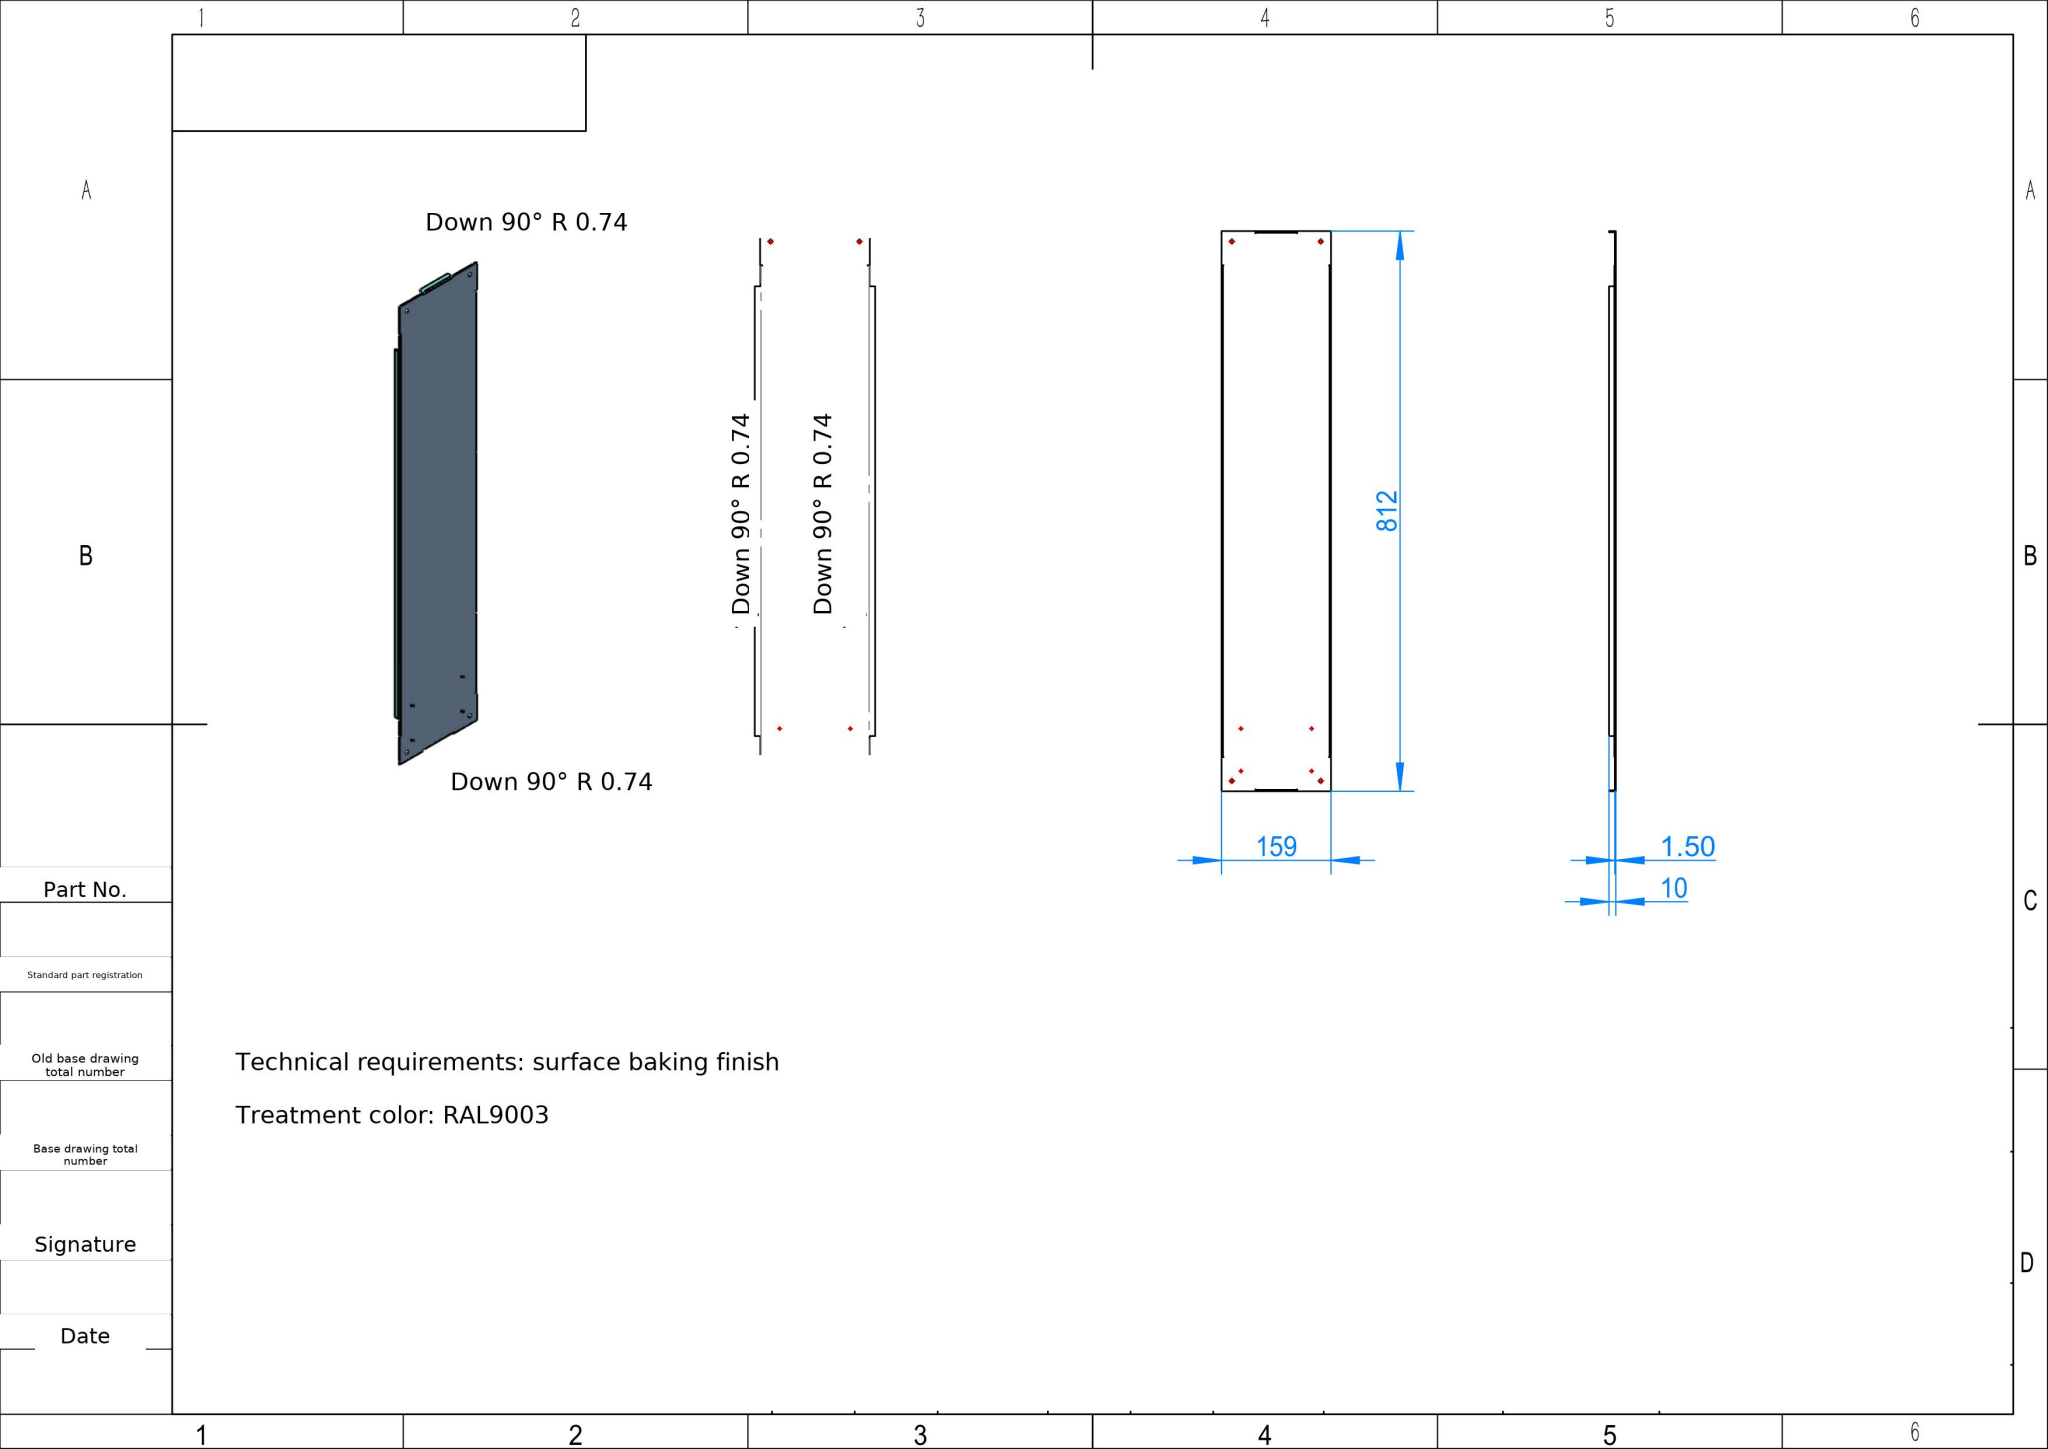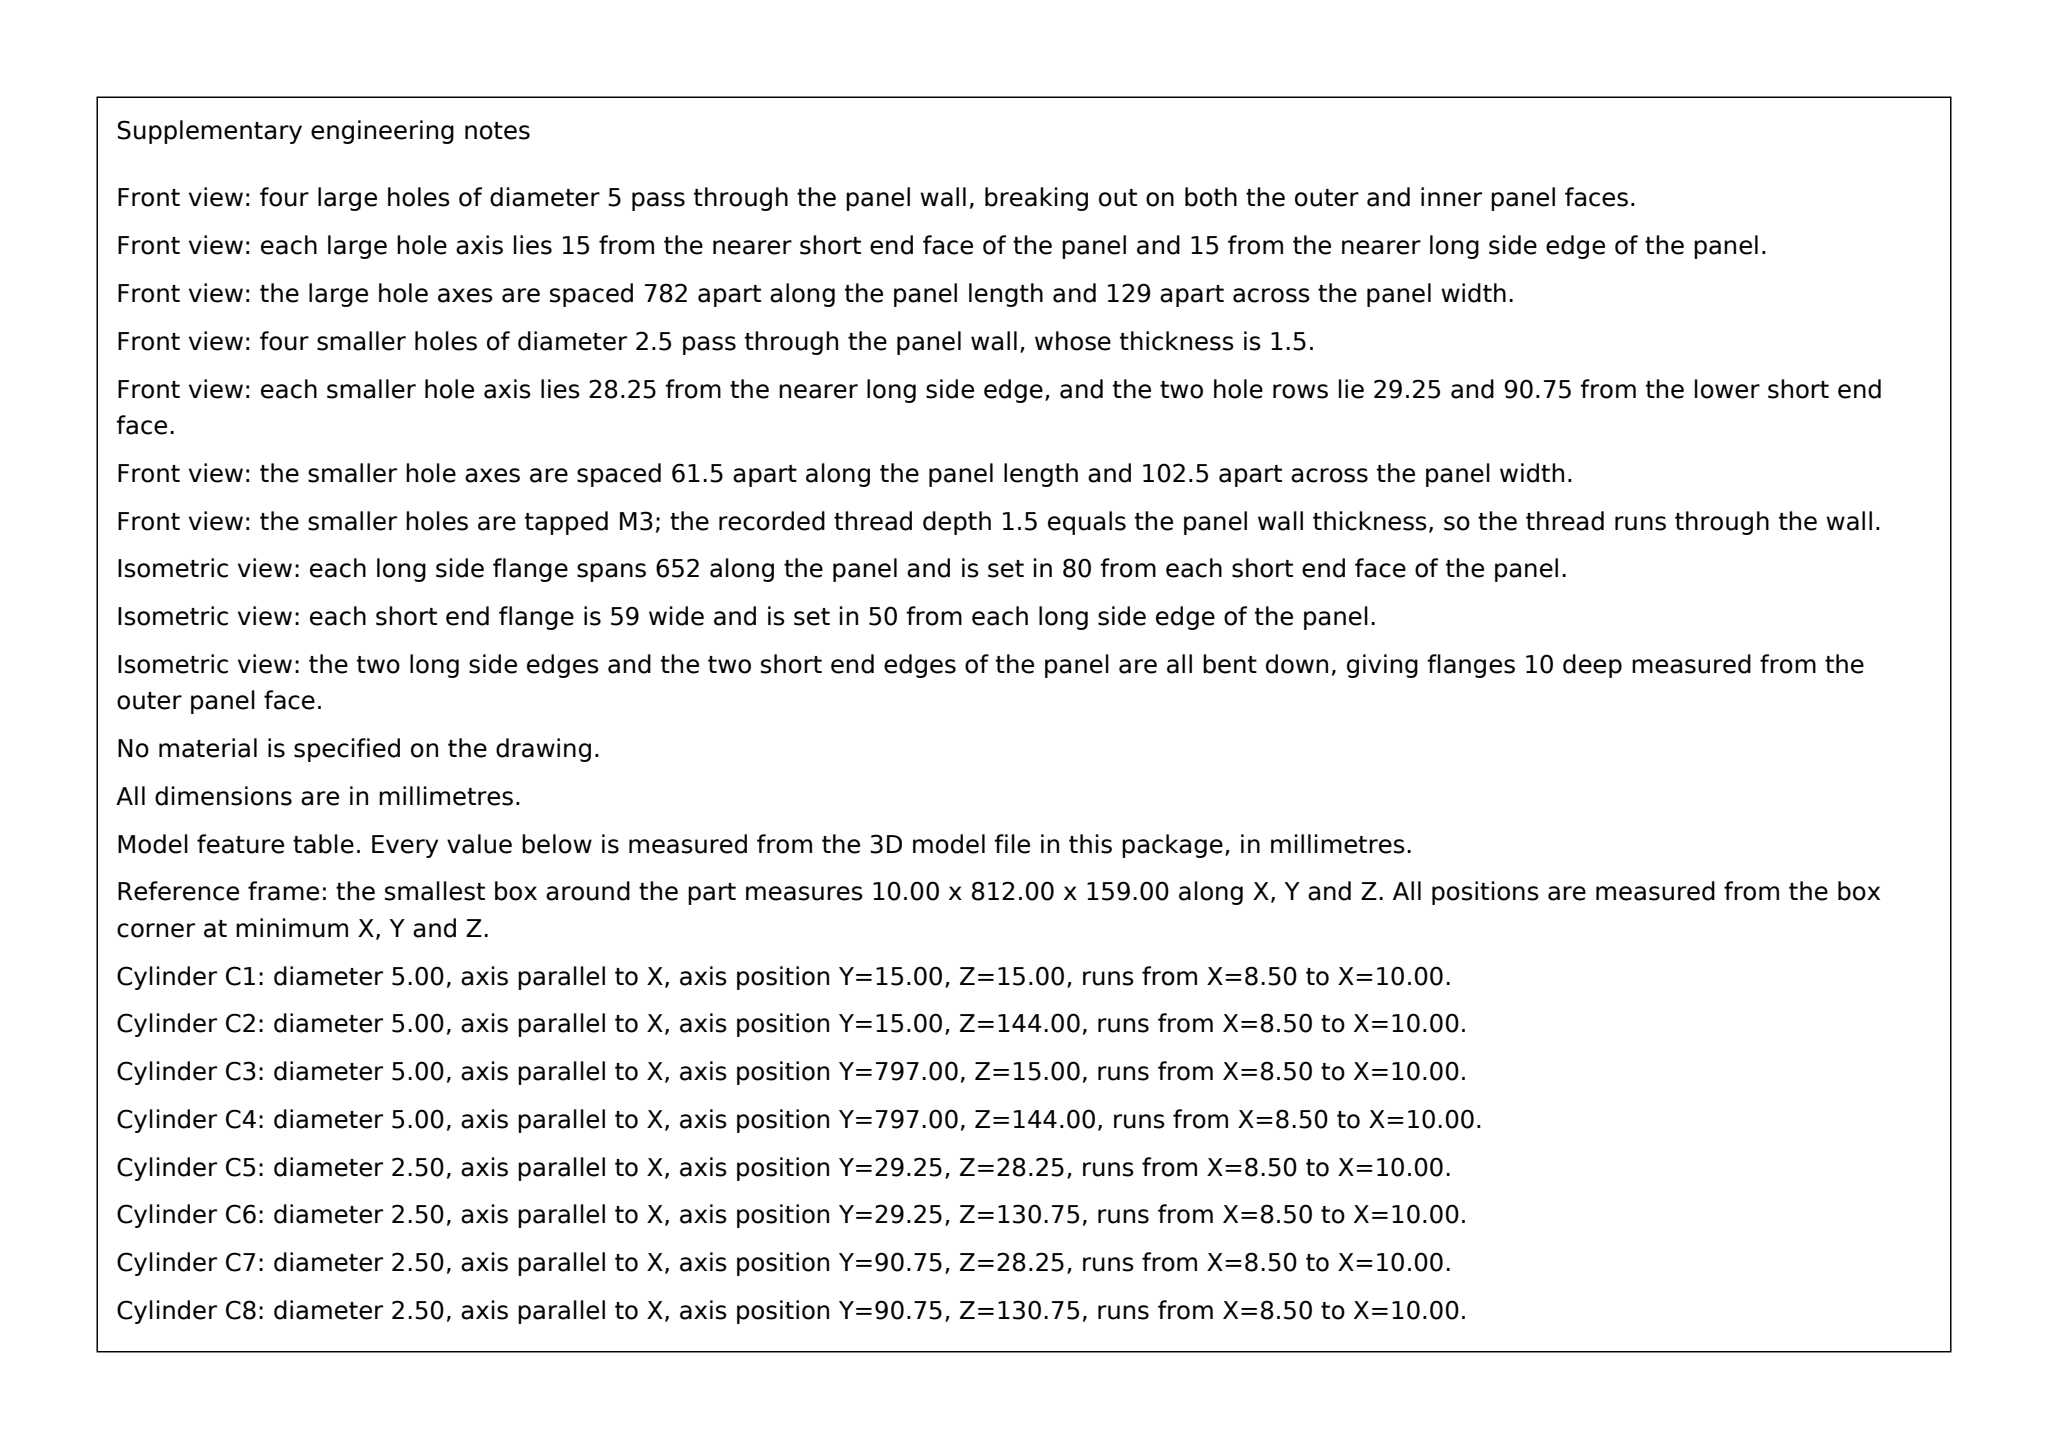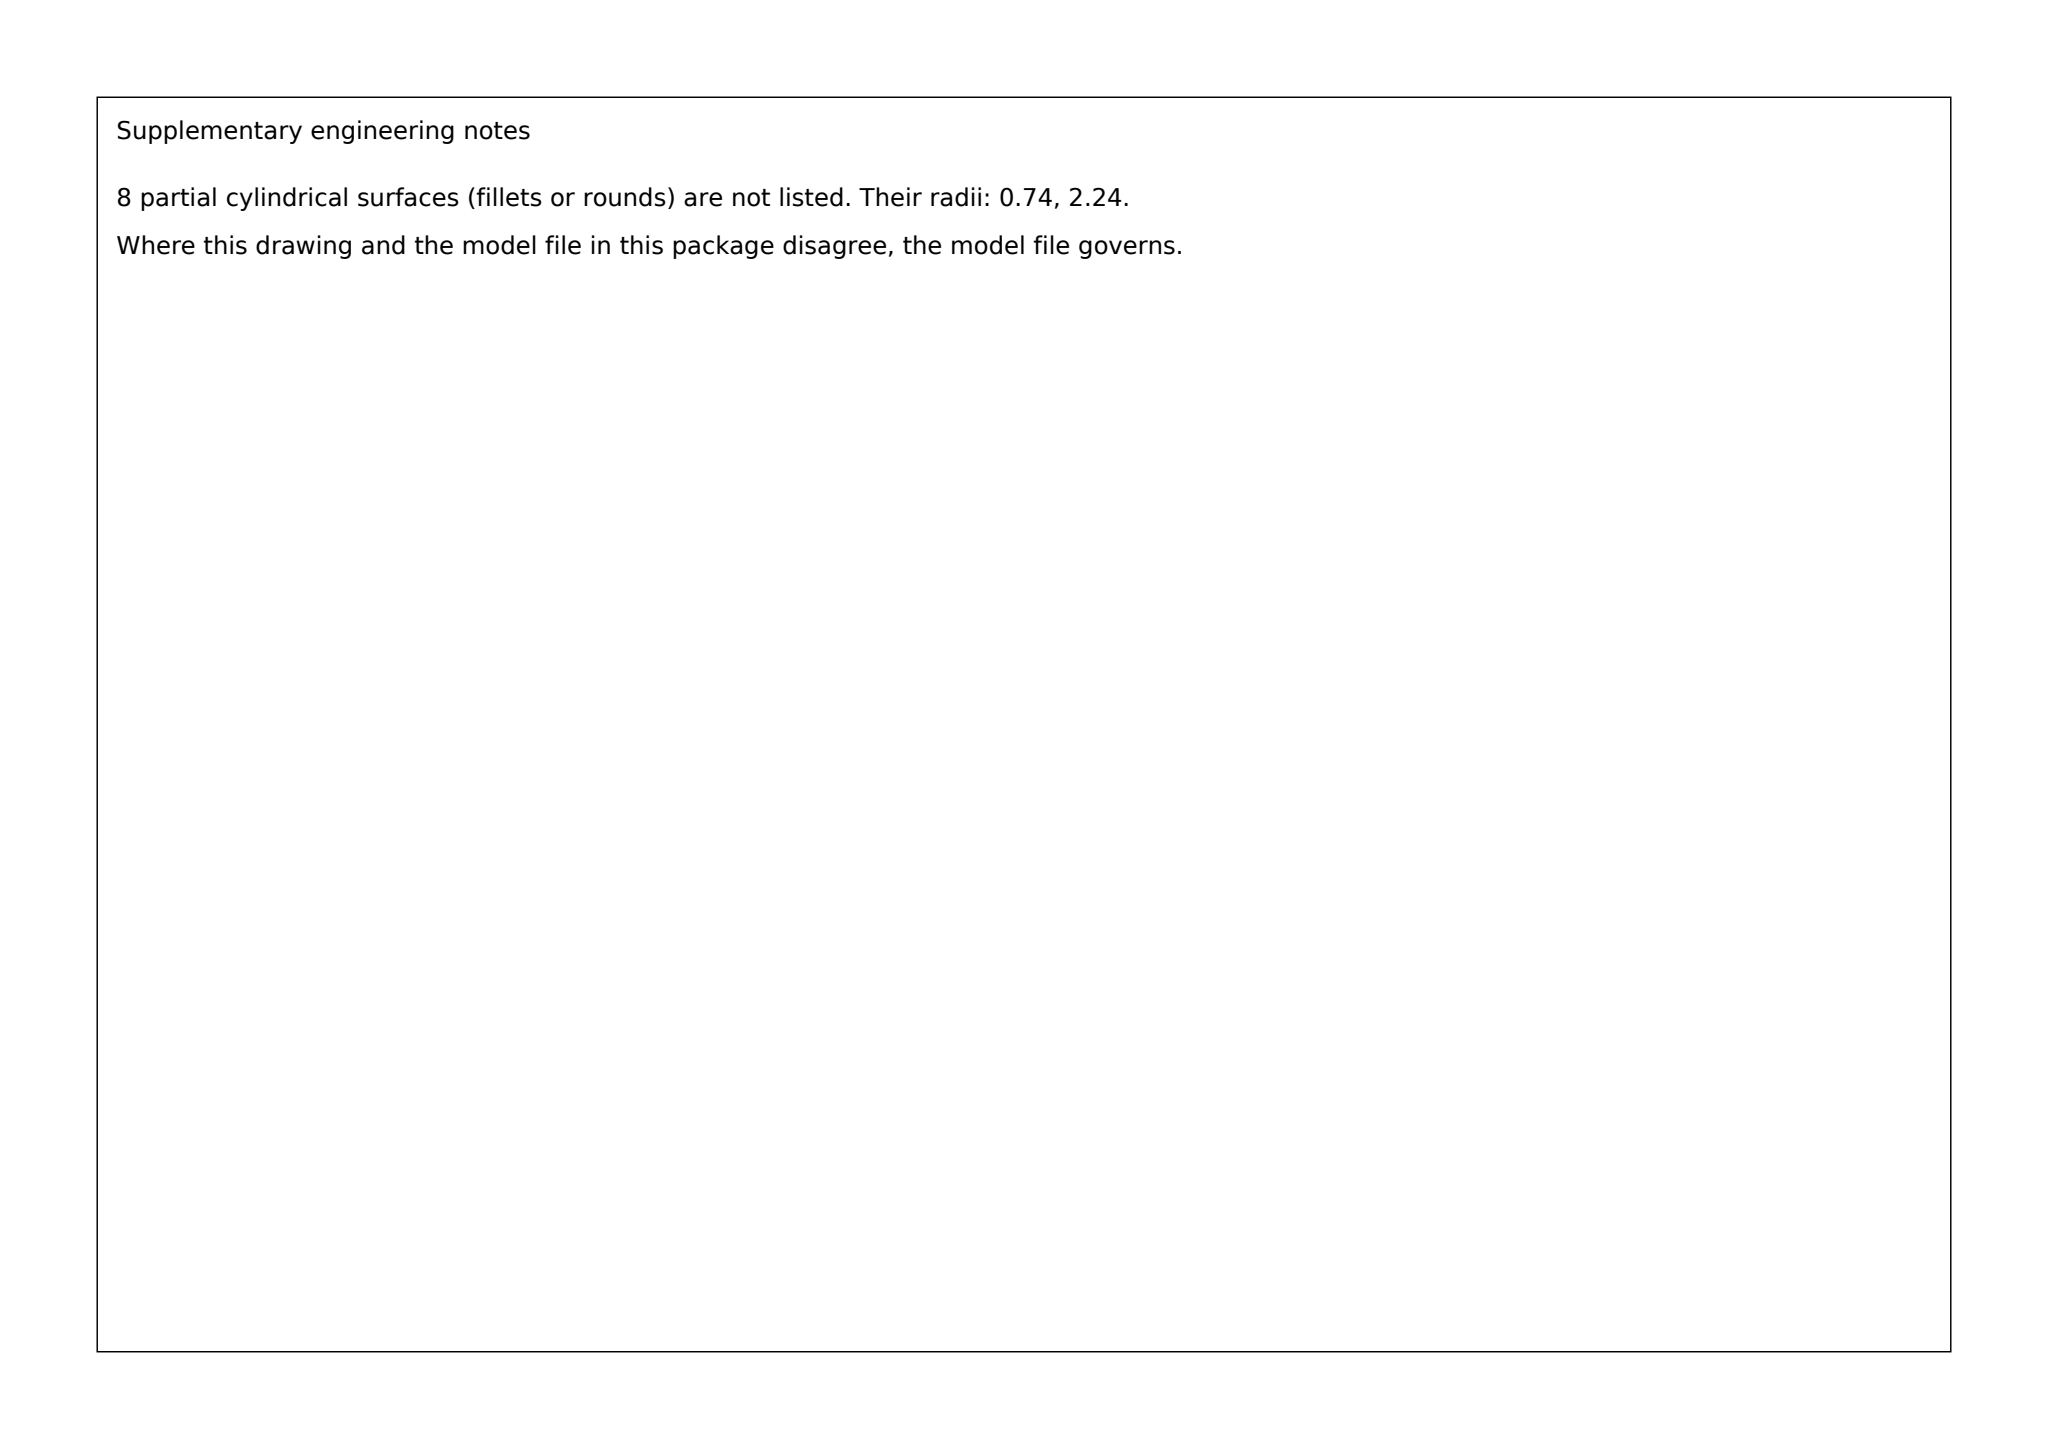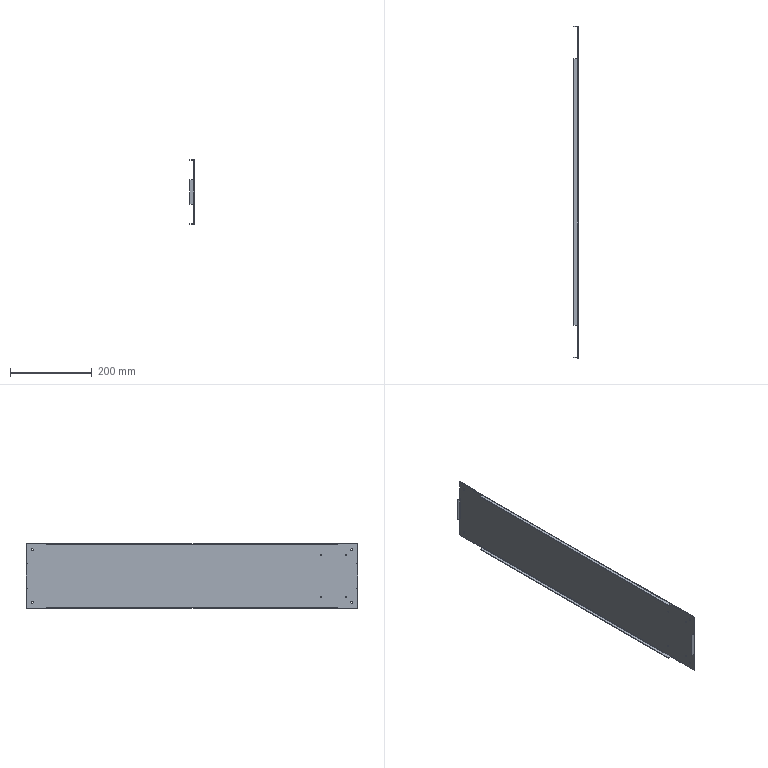Part | SolidWorks | mm | 1 solid | 94 faces | box 10 x 812 x 159 mm | volume 210185 mm3 | plane 70 | cylinder 24 | commonest cylinder face diameters 5 x8 2.5 x8 4.473 x4 1.473 x4
Drawing notes:
4X Ø5.0 THRU IN FLAT FACE | from the solid: cylinders dia 5.0, axis x, length 1.5 (sheet thk), 4 locations
Ø5.0 HOLES: 15 FROM EACH EDGE, 782 CTRS LG X 129 CTRS WD | from the solid: dia5.0 pos (y,z)=(15,15),(15,144),(797,15),(797,144); 812x159 bbox
4X Ø2.5 THRU IN FLAT FACE | from the solid: cylinders dia 2.5, axis x, length 1.5, 4 locations
Ø2.5 CTRS 29.25 & 90.75 FROM END EDGE, 28.25 & 130.75 FROM SIDE | from the solid: dia2.5 pos (y,z)=(29.25/90.75, 28.25/130.75), y=0 & z=0 datum edges
FLANGE RELIEFS: 50-80 & 732-762 FROM END; 50-109 FROM SIDE | from the solid: axis planes y=50,80,732,762 and z=50,109 bounding notch faces
SIDE FLANGES 712 LG, END FLANGES 59 LG, 10 HIGH | from the solid: bend cyl lengths 712 (axis y) & 59 (axis z); bbox x=10
FLAT PATTERN BEND LINES 2.99 FROM EACH OUTER EDGE | from the solid: axis planes y=2.99/809.01 and z=2.99/156.01 (bend tangent faces)